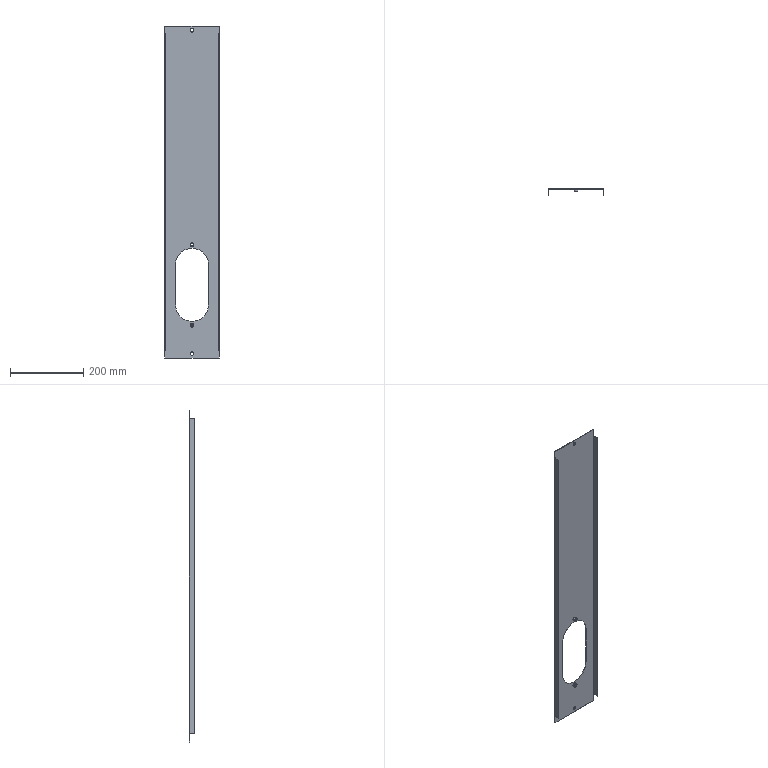Component | SolidWorks | BottomPlateMountingPlate2-1 | 1 solid | 67 faces | volume 172085 mm3 | cylinder 35 | plane 28 | spline 4 | commonest cylinder face diameters 3 x10 7 x6 6 x4 11 x4 8 x4 90 x3 0.2 x2 2.6 x2